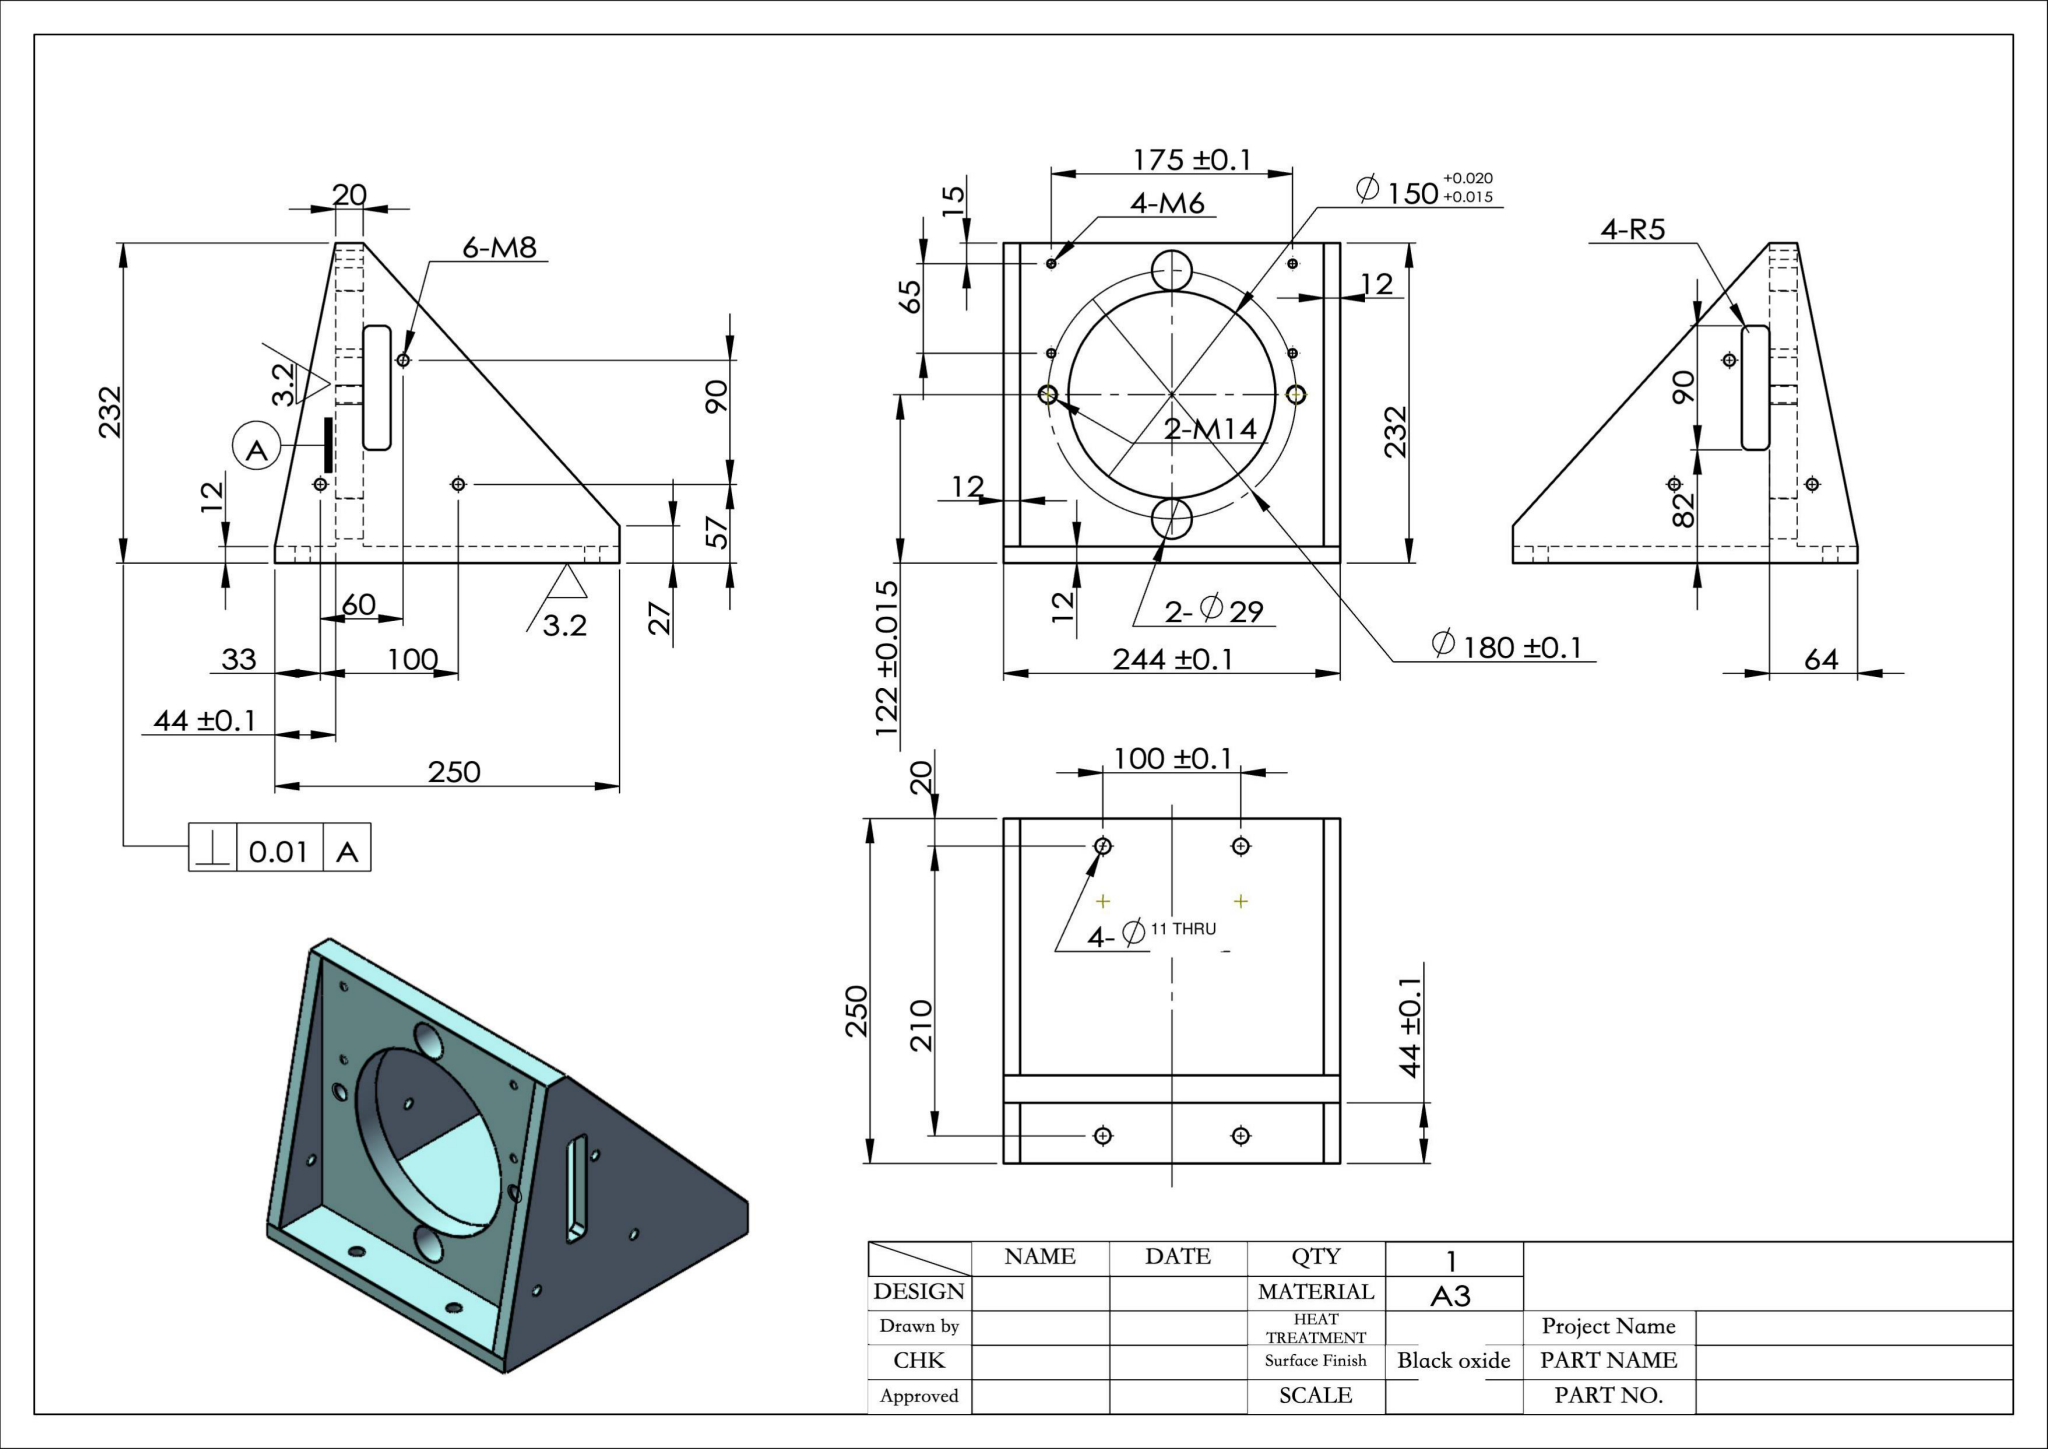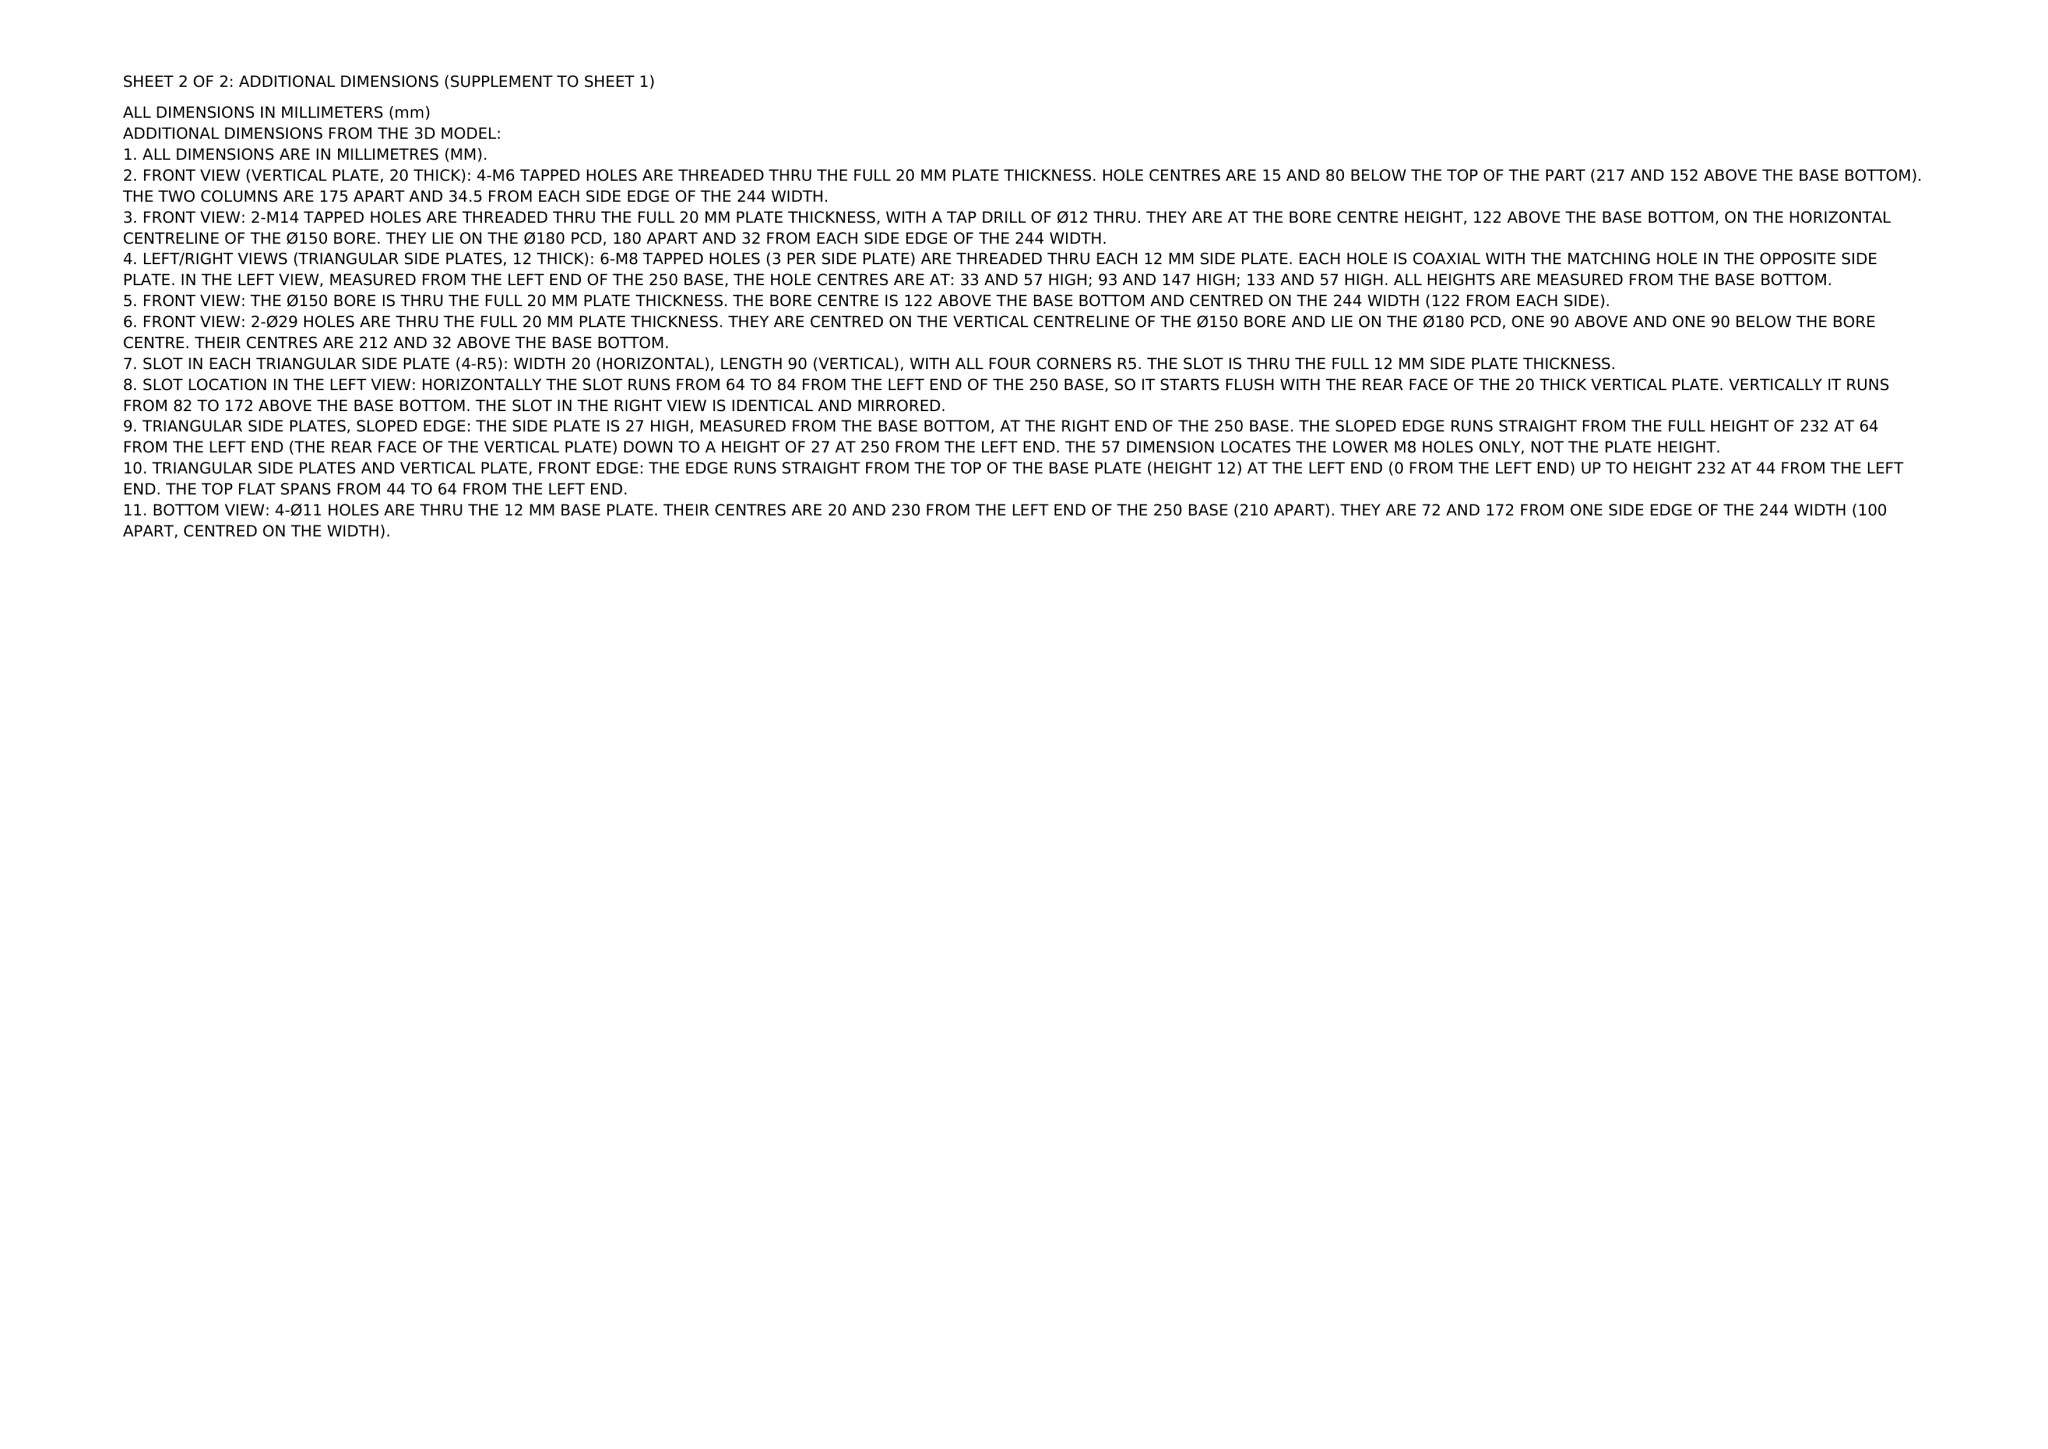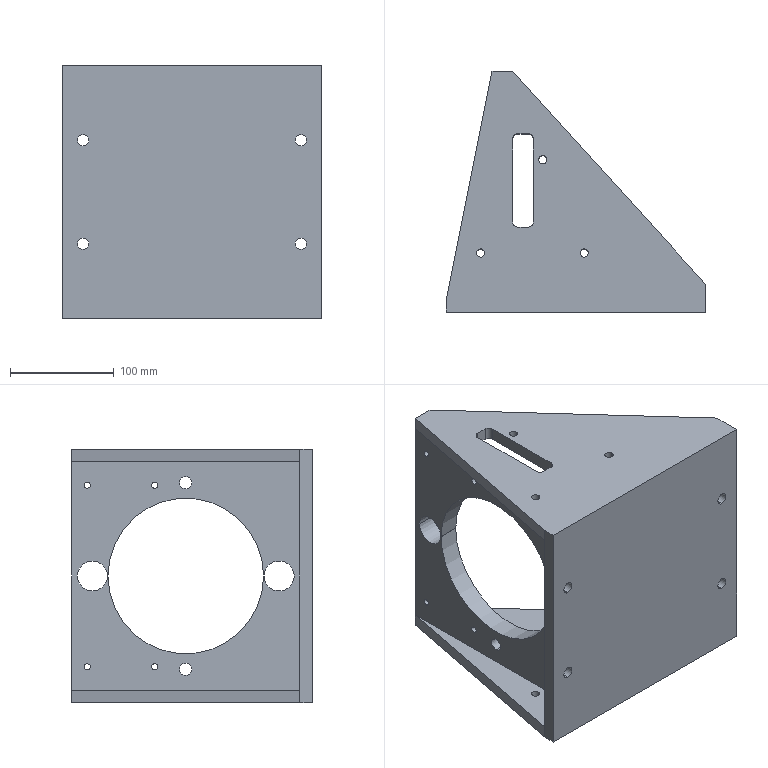Part | NX | mm | 1 solid | 70 faces | box 250 x 232 x 244 mm | volume 2008779 mm3 | cylinder 46 | plane 24 | commonest cylinder face diameters 8 x12 6 x8 11 x8 10 x8 12 x4 29 x4 150 x2